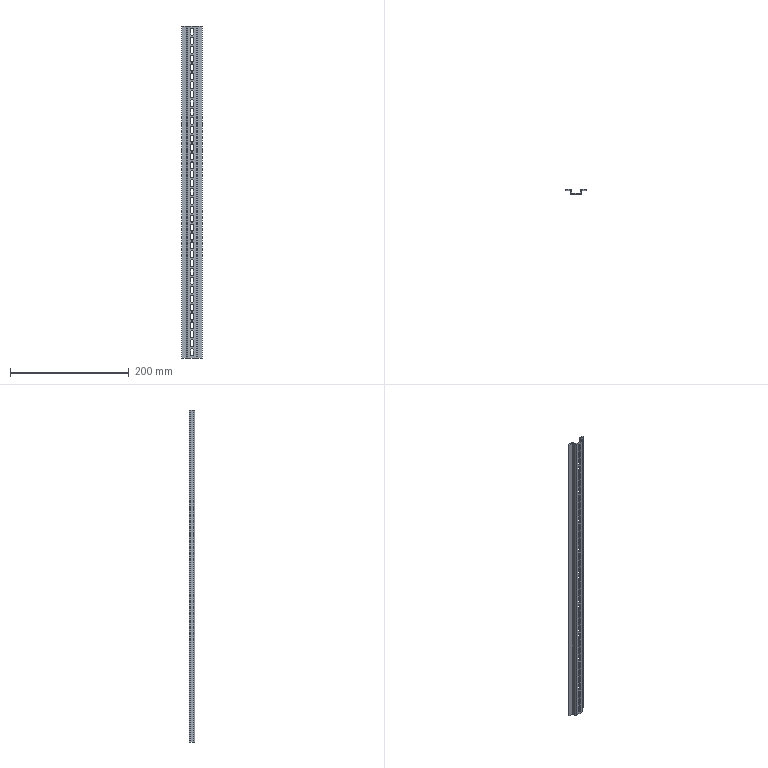Component | SolidWorks | VoltageTerminalRail-1 | 1 solid | 186 faces | volume 37165 mm3 | plane 104 | cylinder 82 | commonest cylinder face diameters 5 x74 4 x4 1 x4